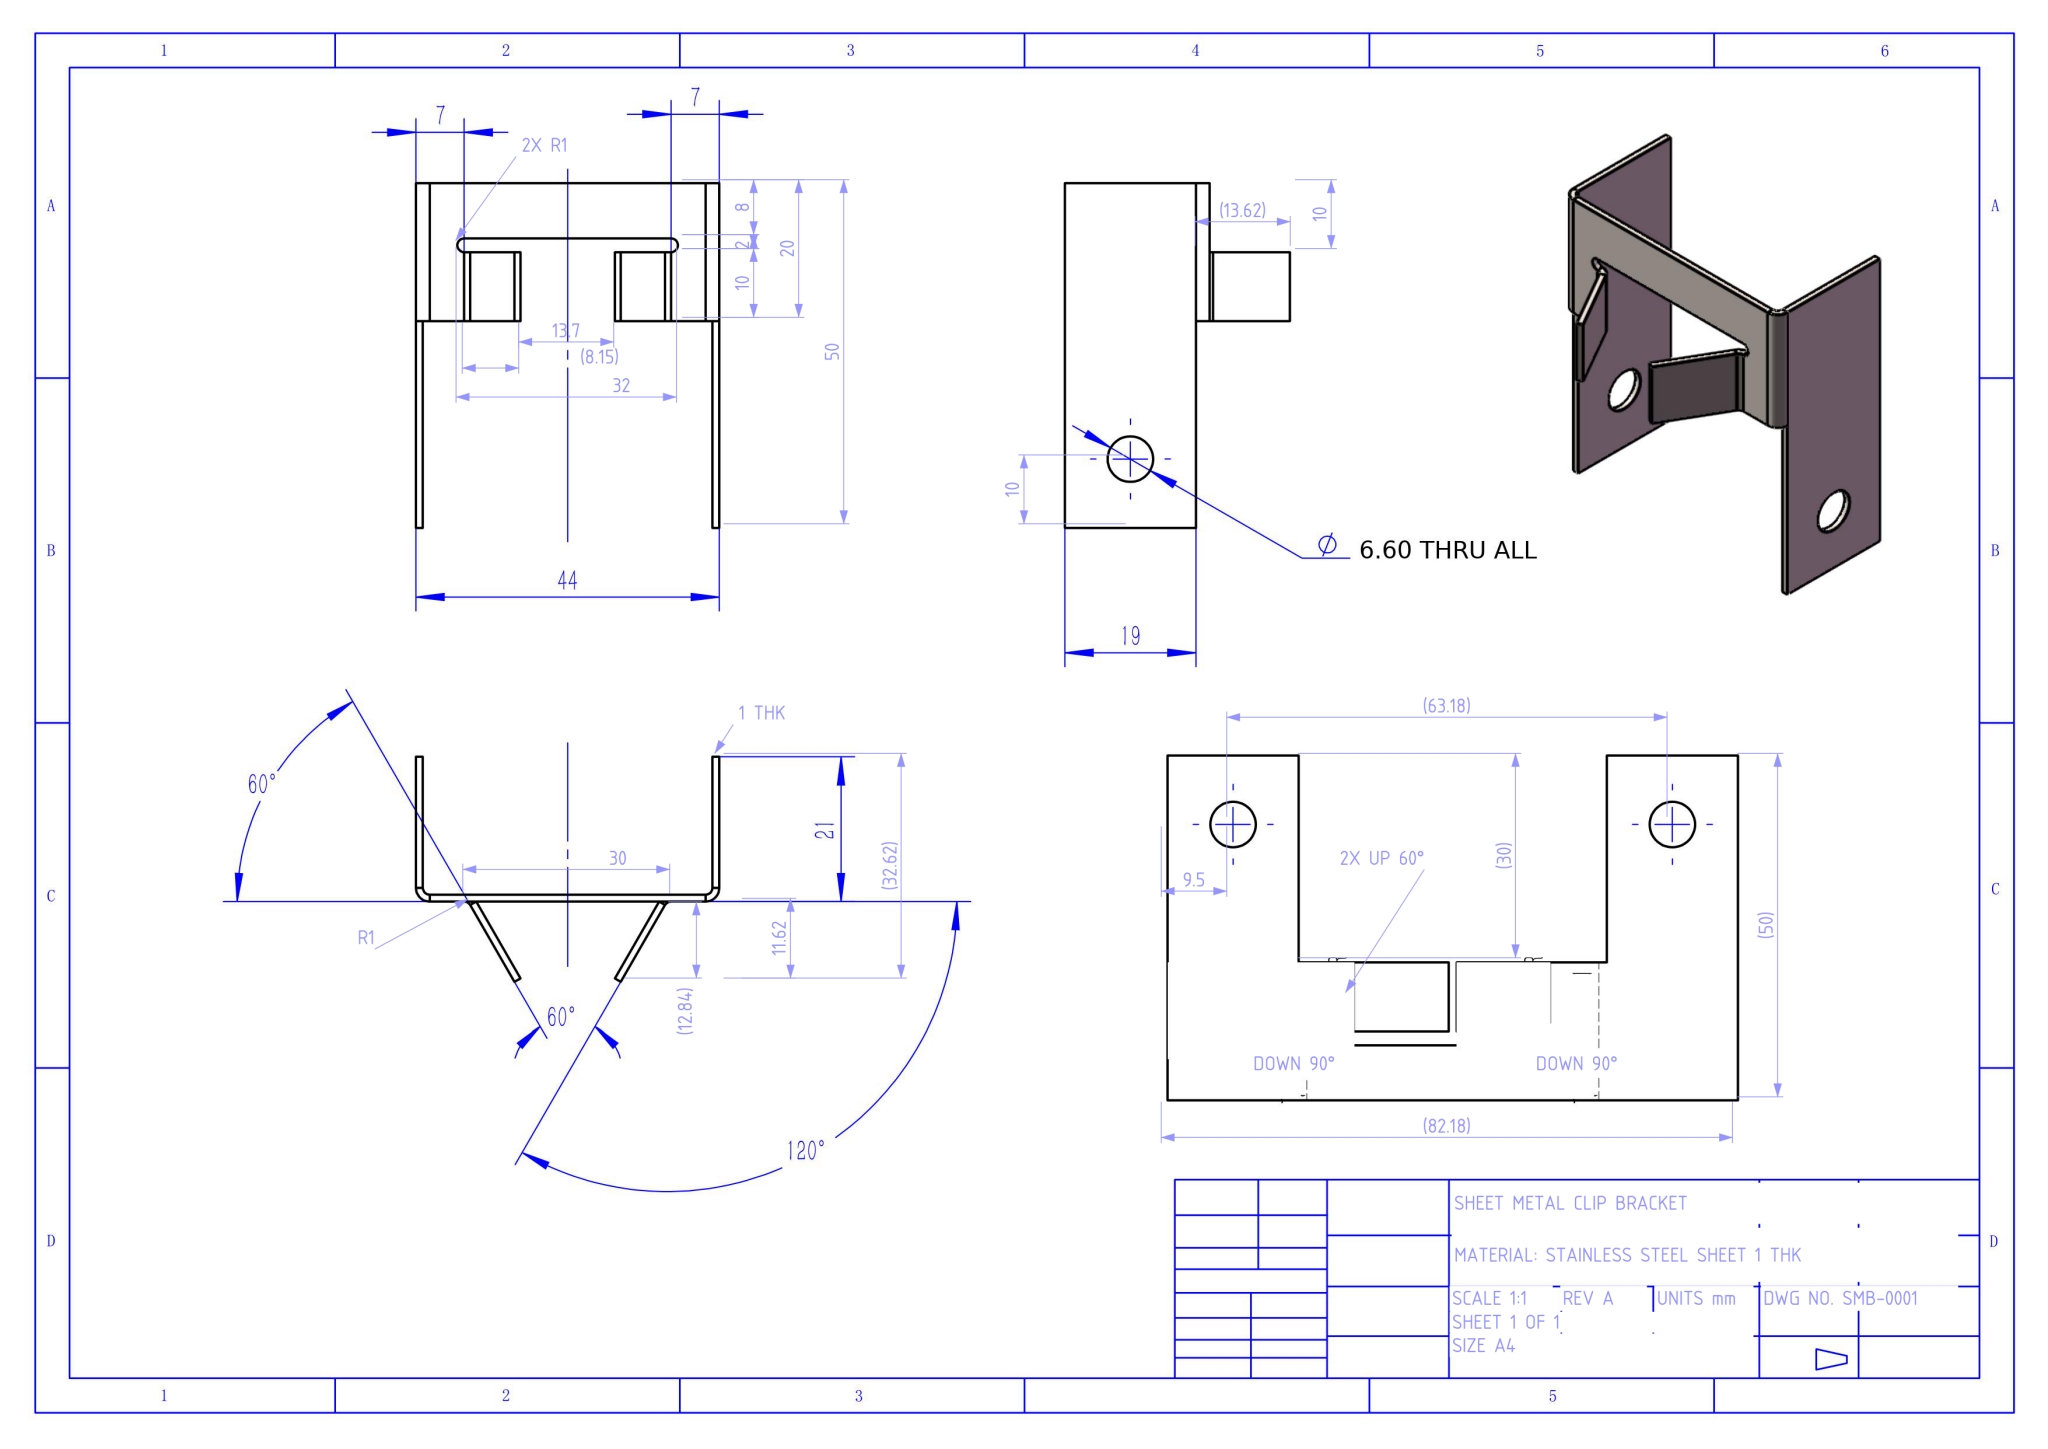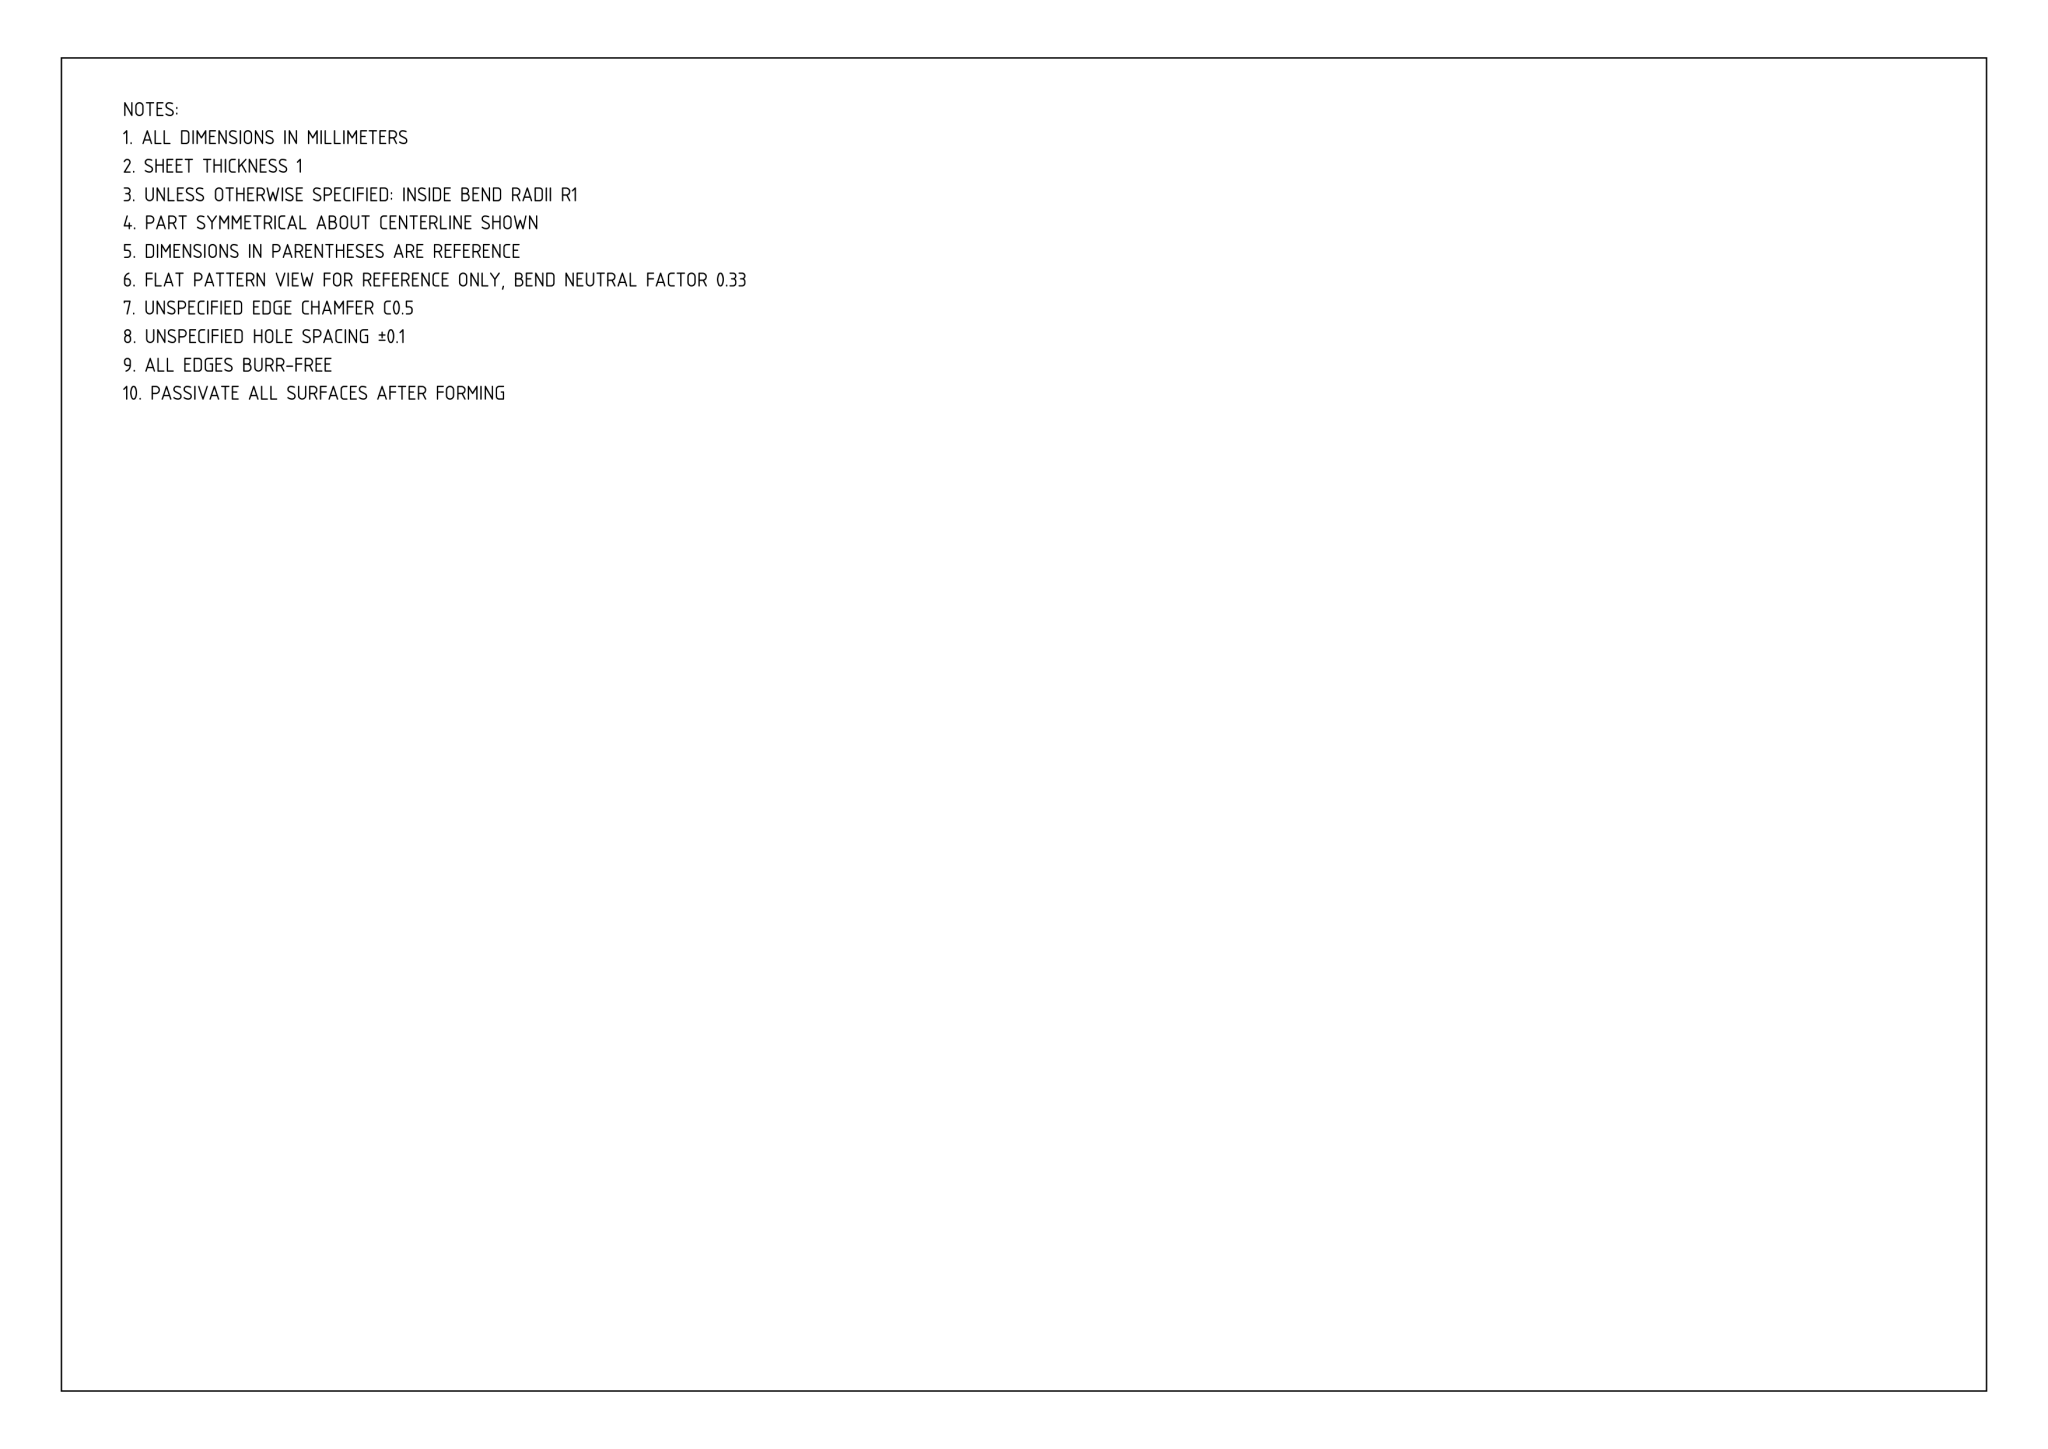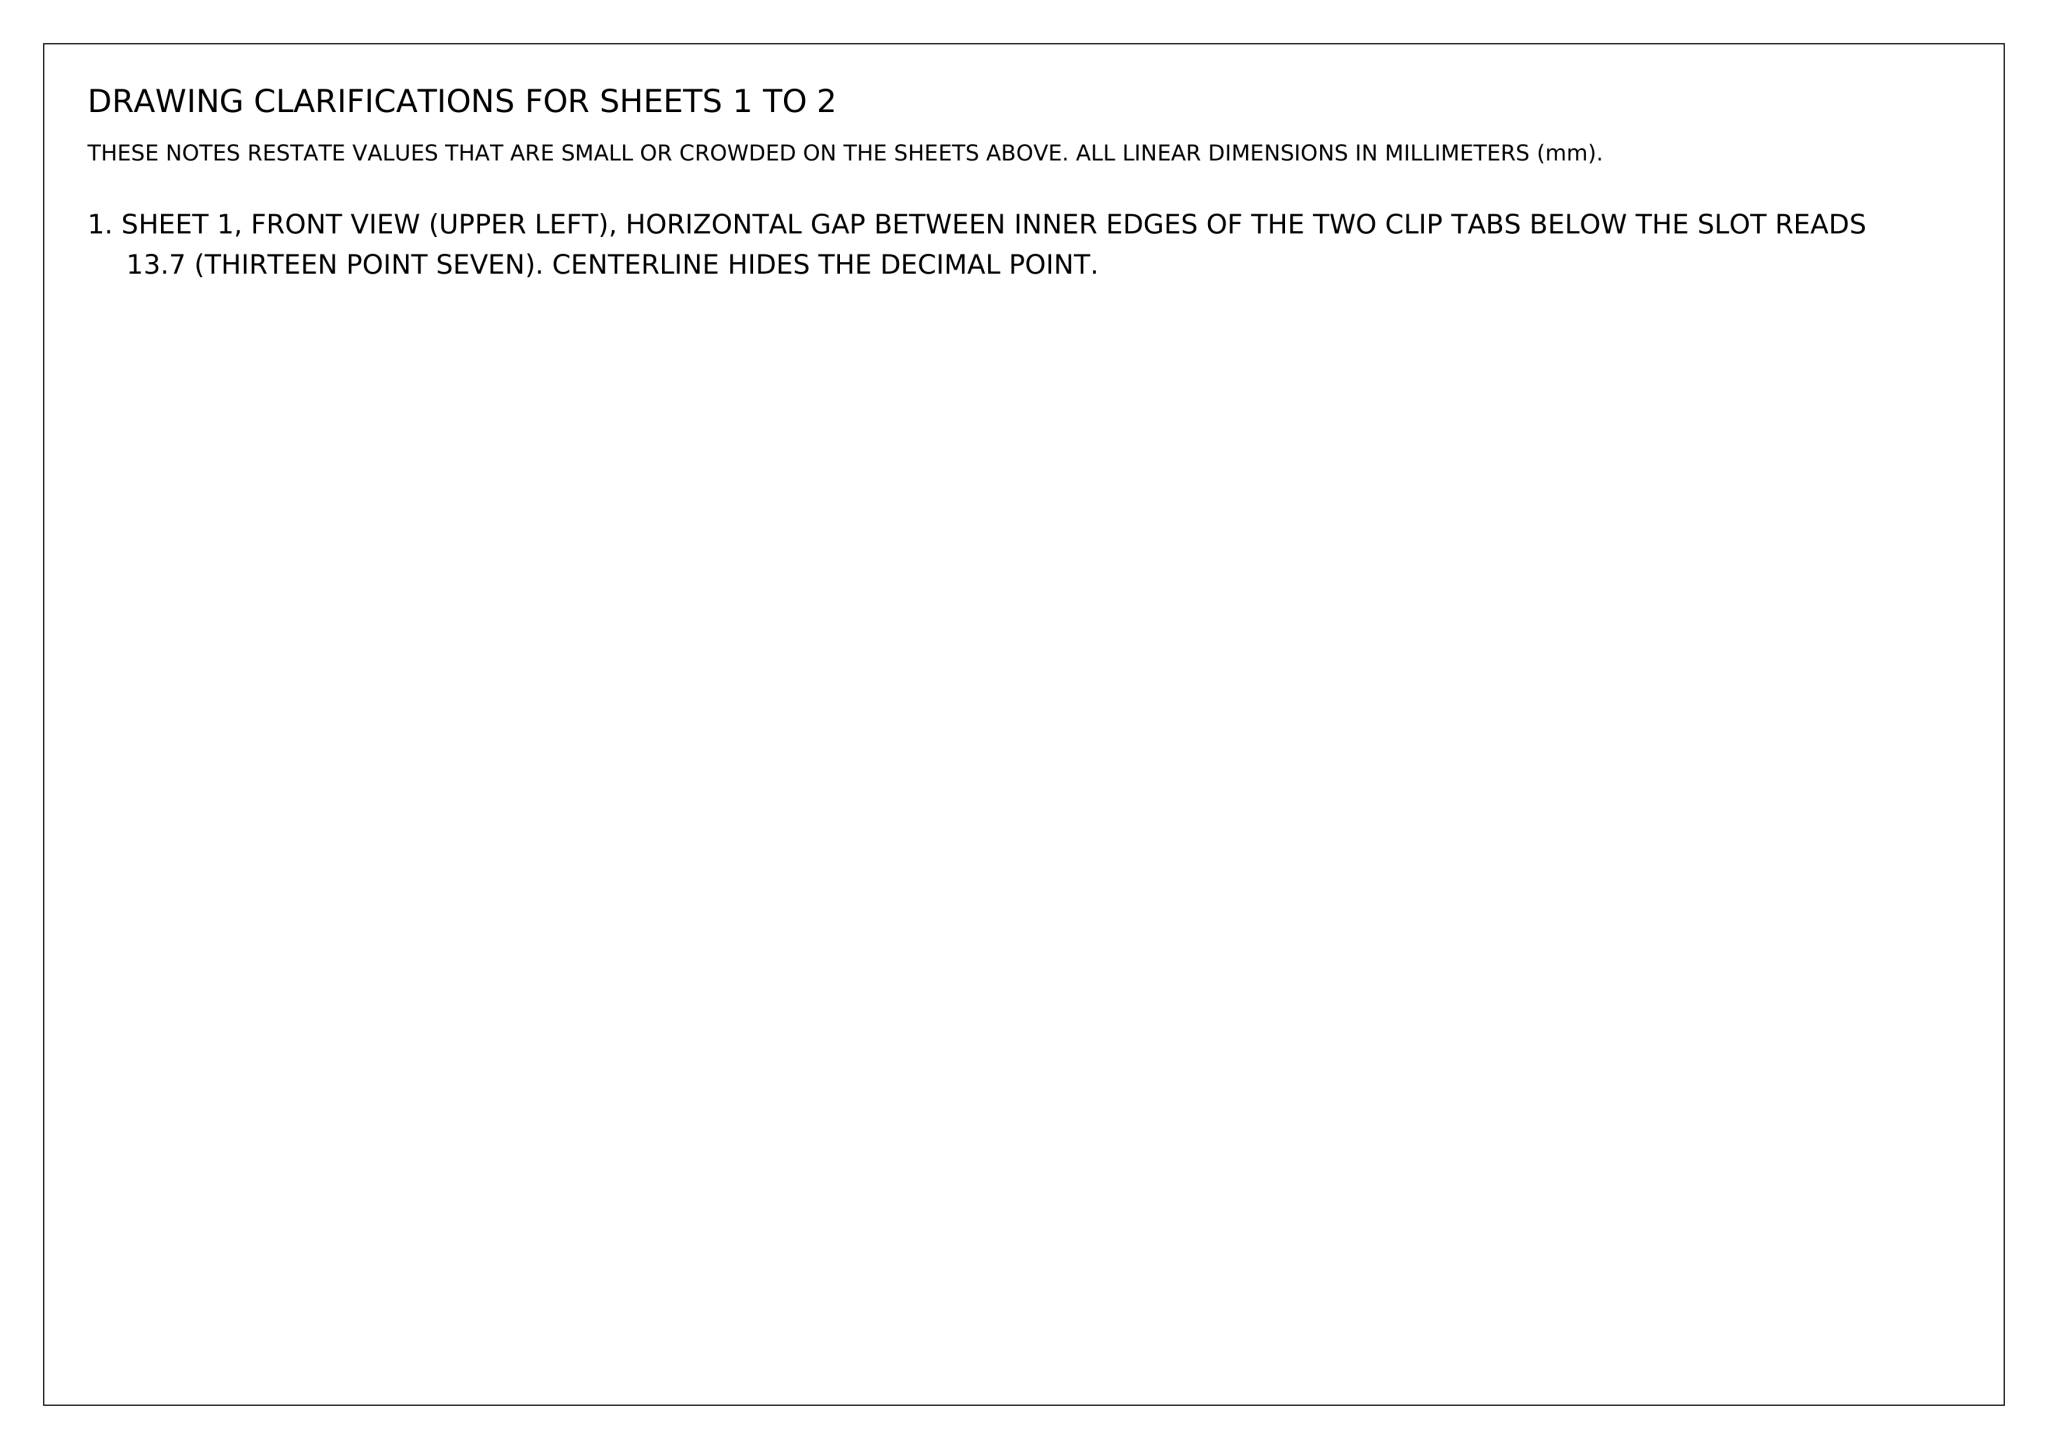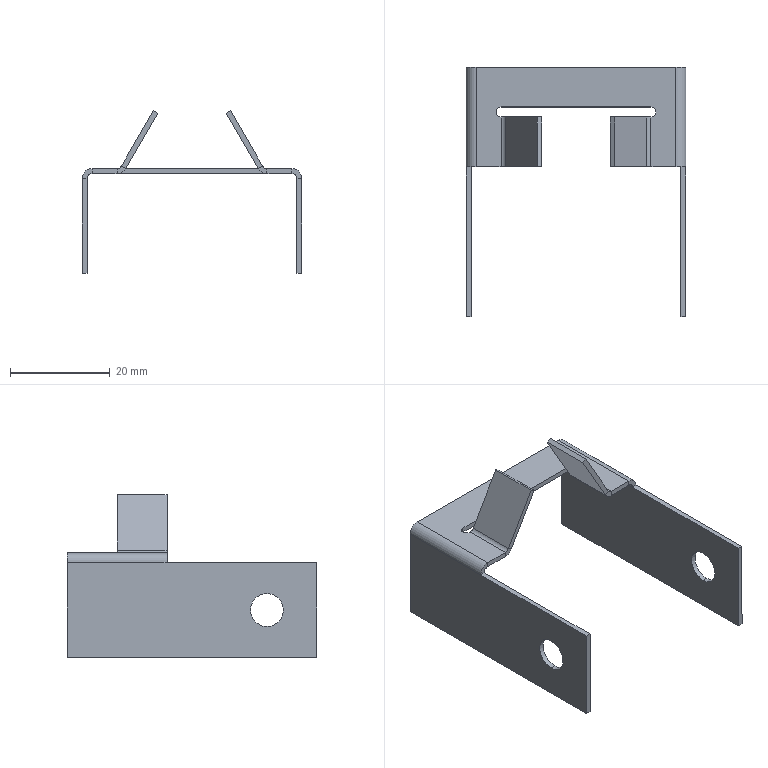Part | NX | mm | 1 solid | 51 faces | box 44 x 50 x 32.62 mm | volume 2651 mm3 | plane 36 | cylinder 15 | commonest cylinder face diameters 2 x7 6.6 x4 4 x4